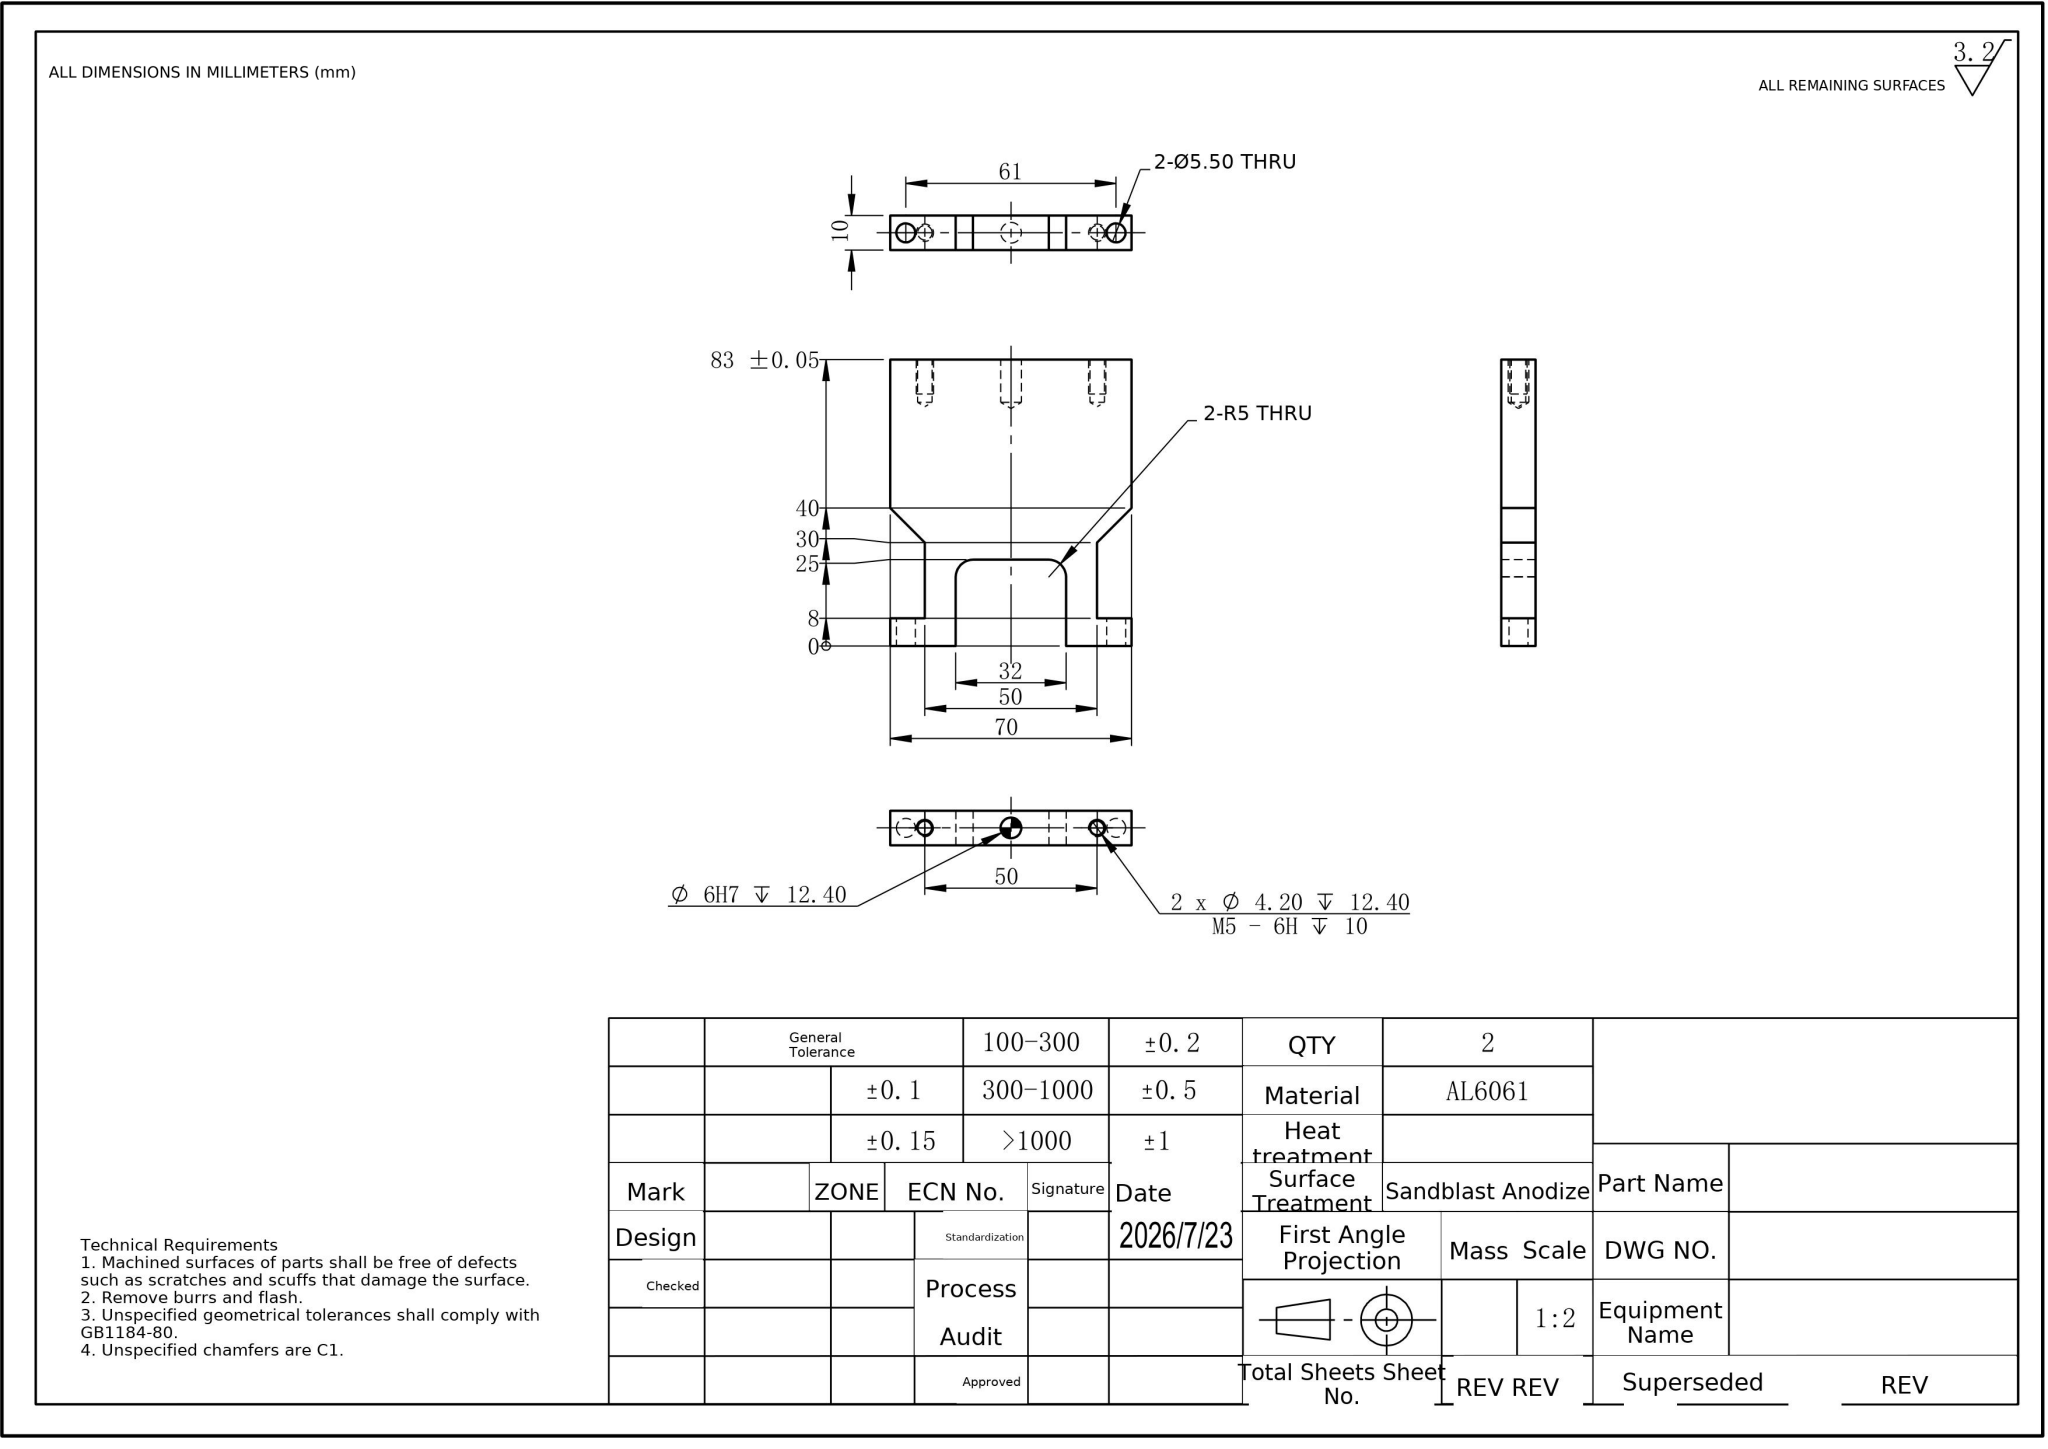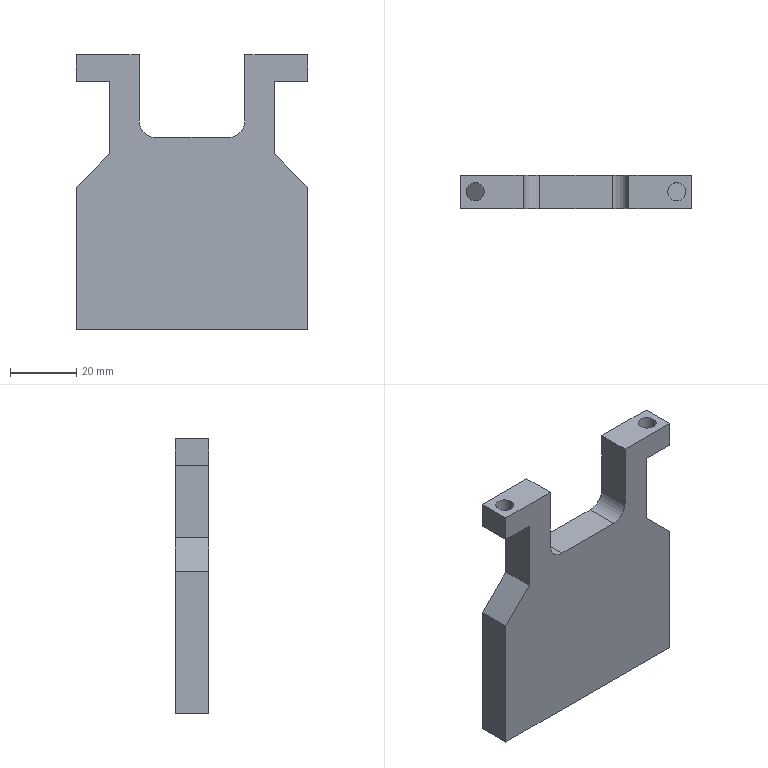Part | NX | mm | 1 solid | 36 faces | box 70 x 10 x 83 mm | volume 43704 mm3 | plane 18 | cylinder 12 | cone 6 | commonest cylinder face diameters 5.5 x4 4.2 x4 6 x2 10 x2